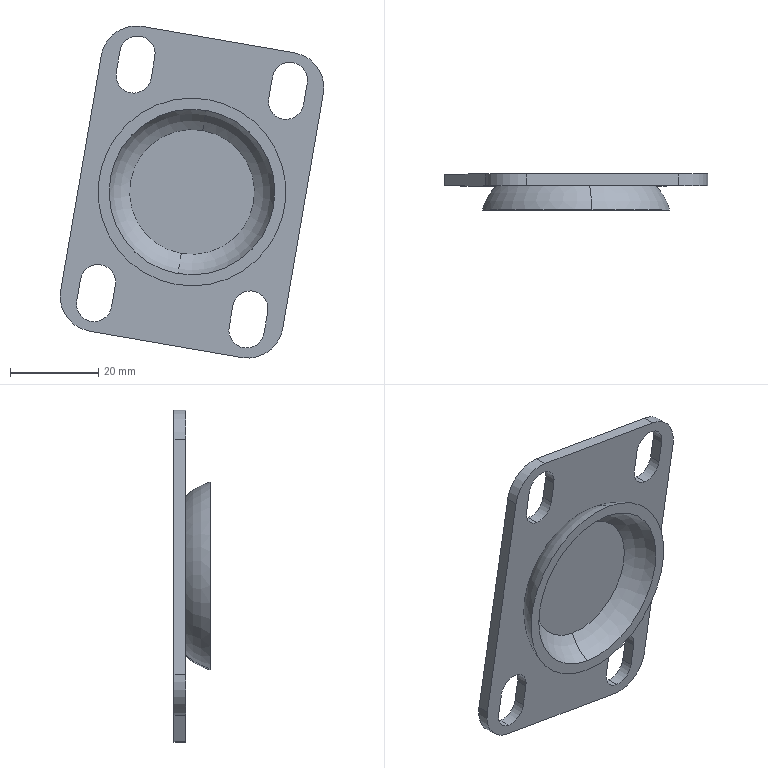Component | SolidWorks | PC-CAJ-P08-1_Rueda 2 in AZUL-1_Pieza2-1 | 1 solid | 39 faces | volume 10226 mm3 | cylinder 18 | plane 17 | torus 4 | commonest cylinder face diameters 8 x12 16 x4 1 x2 | material Plain Carbon Steel